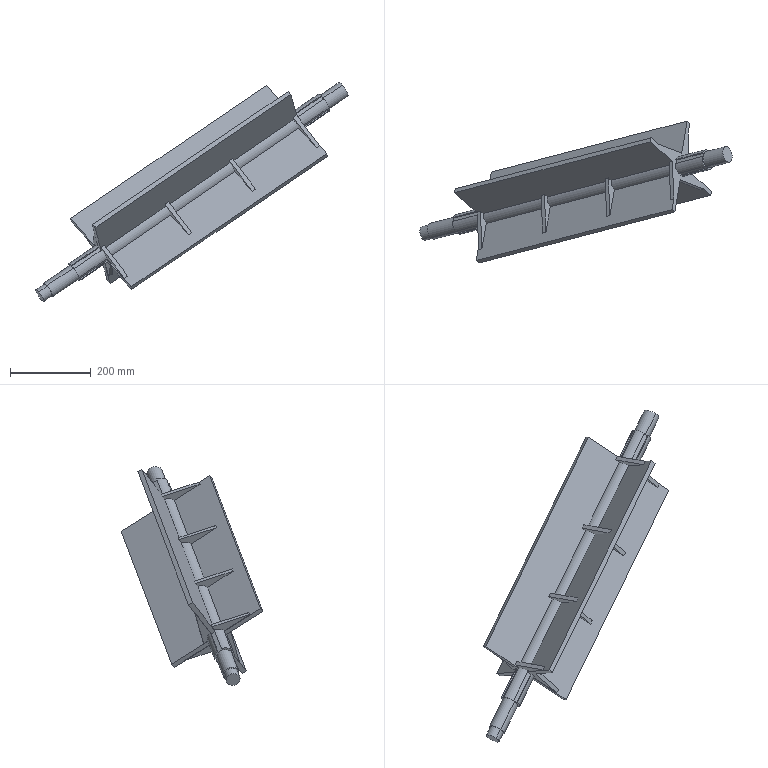Component | SolidWorks | CutterAxisII-1 | 1 solid | 116 faces | volume 4920902 mm3 | plane 90 | cylinder 26 | commonest cylinder face diameters 50 x20 40 x4 35 x2